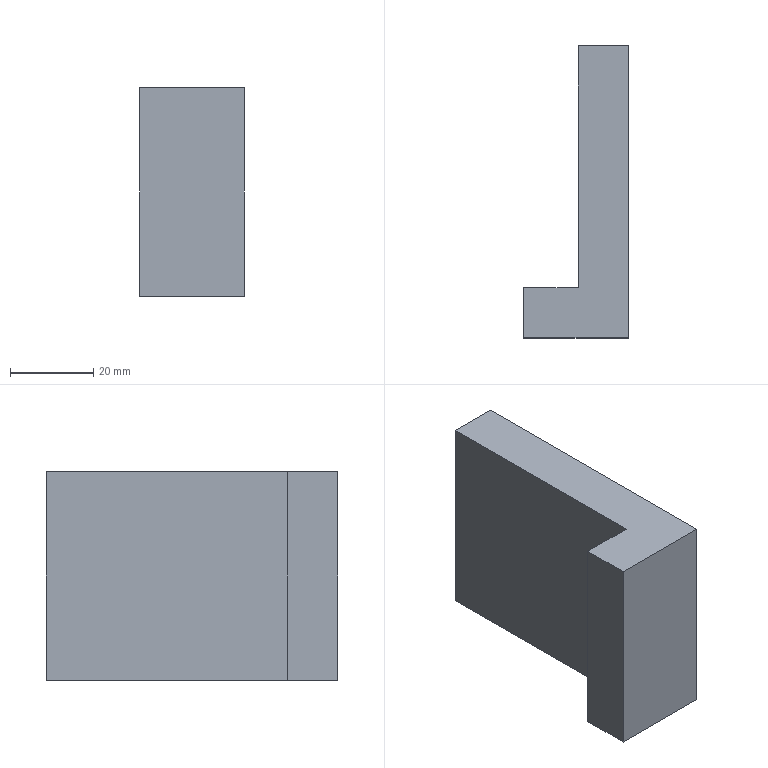Component | NX | CLAMP_PLATE_2 | 1 solid | 14 faces | box 25 x 70 x 50 mm | volume 49383 mm3 | plane 8 | cone 4 | cylinder 2 | commonest cylinder face diameters 5 x2
STEP:
#1=CARTESIAN_POINT('',(0.,0.,0.));
#2=DIRECTION('',(0.,0.,1.));
#3=DIRECTION('',(1.,0.,0.));
#4=AXIS2_PLACEMENT_3D('',#1,#2,#3);
#5=CARTESIAN_POINT('',(117.866,129.757,24.466));
#6=VERTEX_POINT('',#5);
#7=CARTESIAN_POINT('',(117.866,71.757,24.466));
#8=VERTEX_POINT('',#7);
#9=CARTESIAN_POINT('',(117.866,129.757,24.466));
#10=DIRECTION('',(-0.,-1.,0.));
#11=VECTOR('',#10,1.);
#12=LINE('',#9,#11);
#13=CARTESIAN_POINT('',(117.866,71.757,24.466));
#14=DIRECTION('',(-1.,0.,0.));
#15=DIRECTION('',(-0.,-1.,0.));
#16=AXIS2_PLACEMENT_3D('',#13,#14,#15);
#17=PLANE('',#16);
#18=CARTESIAN_POINT('',(-58.,0.));
#19=DIRECTION('',(1.,0.));
#20=VECTOR('',#19,1.);
#21=LINE('',#18,#20);
#22=(GEOMETRIC_REPRESENTATION_CONTEXT(2)PARAMETRIC_REPRESENTATION_CONTEXT()REPRESENTATION_CONTEXT('',''));
#23=DEFINITIONAL_REPRESENTATION('',(#21),#22);
#24=PCURVE('',#17,#23);
#25=CARTESIAN_POINT('',(129.866,59.757,24.466));
#26=DIRECTION('',(0.,0.,1.));
#27=DIRECTION('',(0.,1.,0.));
#28=AXIS2_PLACEMENT_3D('',#25,#26,#27);
#29=PLANE('',#28);
#30=CARTESIAN_POINT('',(70.,12.));
#31=DIRECTION('',(-1.,0.));
#32=VECTOR('',#31,1.);
#33=LINE('',#30,#32);
#34=(GEOMETRIC_REPRESENTATION_CONTEXT(2)PARAMETRIC_REPRESENTATION_CONTEXT()REPRESENTATION_CONTEXT('',''));
#35=DEFINITIONAL_REPRESENTATION('',(#33),#34);
#36=PCURVE('',#29,#35);
#37=SURFACE_CURVE('',#12,(#24,#36),.PCURVE_S1.);
#38=EDGE_CURVE('',#6,#8,#37,.T.);
#39=ORIENTED_EDGE('',*,*,#38,.T.);
#40=CARTESIAN_POINT('',(117.866,71.757,74.466));
#41=VERTEX_POINT('',#40);
#42=CARTESIAN_POINT('',(117.866,71.757,24.466));
#43=DIRECTION('',(0.,0.,1.));
#44=VECTOR('',#43,1.);
#45=LINE('',#42,#44);
#46=CARTESIAN_POINT('',(0.,0.));
#47=DIRECTION('',(0.,1.));
#48=VECTOR('',#47,1.);
#49=LINE('',#46,#48);
#50=(GEOMETRIC_REPRESENTATION_CONTEXT(2)PARAMETRIC_REPRESENTATION_CONTEXT()REPRESENTATION_CONTEXT('',''));
#51=DEFINITIONAL_REPRESENTATION('',(#49),#50);
#52=PCURVE('',#17,#51);
#53=CARTESIAN_POINT('',(117.866,71.757,24.466));
#54=DIRECTION('',(0.,1.,0.));
#55=DIRECTION('',(-1.,0.,0.));
#56=AXIS2_PLACEMENT_3D('',#53,#54,#55);
#57=PLANE('',#56);
#58=CARTESIAN_POINT('',(0.,0.));
#59=DIRECTION('',(0.,1.));
#60=VECTOR('',#59,1.);
#61=LINE('',#58,#60);
#62=(GEOMETRIC_REPRESENTATION_CONTEXT(2)PARAMETRIC_REPRESENTATION_CONTEXT()REPRESENTATION_CONTEXT('',''));
#63=DEFINITIONAL_REPRESENTATION('',(#61),#62);
#64=PCURVE('',#57,#63);
#65=SURFACE_CURVE('',#45,(#52,#64),.PCURVE_S1.);
#66=EDGE_CURVE('',#8,#41,#65,.T.);
#67=ORIENTED_EDGE('',*,*,#66,.T.);
#68=CARTESIAN_POINT('',(117.866,129.757,74.466));
#69=VERTEX_POINT('',#68);
#70=CARTESIAN_POINT('',(117.866,71.757,74.466));
#71=DIRECTION('',(-0.,-1.,0.));
#72=VECTOR('',#71,1.);
#73=LINE('',#70,#72);
#74=CARTESIAN_POINT('',(0.,50.));
#75=DIRECTION('',(1.,0.));
#76=VECTOR('',#75,1.);
#77=LINE('',#74,#76);
#78=(GEOMETRIC_REPRESENTATION_CONTEXT(2)PARAMETRIC_REPRESENTATION_CONTEXT()REPRESENTATION_CONTEXT('',''));
#79=DEFINITIONAL_REPRESENTATION('',(#77),#78);
#80=PCURVE('',#17,#79);
#81=CARTESIAN_POINT('',(129.866,59.757,74.466));
#82=DIRECTION('',(0.,0.,1.));
#83=DIRECTION('',(0.,1.,0.));
#84=AXIS2_PLACEMENT_3D('',#81,#82,#83);
#85=PLANE('',#84);
#86=CARTESIAN_POINT('',(12.,12.));
#87=DIRECTION('',(-1.,0.));
#88=VECTOR('',#87,1.);
#89=LINE('',#86,#88);
#90=(GEOMETRIC_REPRESENTATION_CONTEXT(2)PARAMETRIC_REPRESENTATION_CONTEXT()REPRESENTATION_CONTEXT('',''));
#91=DEFINITIONAL_REPRESENTATION('',(#89),#90);
#92=PCURVE('',#85,#91);
#93=SURFACE_CURVE('',#73,(#80,#92),.PCURVE_S1.);
#94=EDGE_CURVE('',#69,#41,#93,.T.);
#95=ORIENTED_EDGE('',*,*,#94,.F.);
#96=CARTESIAN_POINT('',(117.866,129.757,24.466));
#97=DIRECTION('',(0.,0.,1.));
#98=VECTOR('',#97,1.);
#99=LINE('',#96,#98);
#100=CARTESIAN_POINT('',(-58.,0.));
#101=DIRECTION('',(0.,1.));
#102=VECTOR('',#101,1.);
#103=LINE('',#100,#102);
#104=(GEOMETRIC_REPRESENTATION_CONTEXT(2)PARAMETRIC_REPRESENTATION_CONTEXT()REPRESENTATION_CONTEXT('',''));
#105=DEFINITIONAL_REPRESENTATION('',(#103),#104);
#106=PCURVE('',#17,#105);
#107=CARTESIAN_POINT('',(129.866,129.757,24.466));
#108=DIRECTION('',(0.,1.,0.));
#109=DIRECTION('',(-1.,0.,0.));
#110=AXIS2_PLACEMENT_3D('',#107,#108,#109);
#111=PLANE('',#110);
#112=CARTESIAN_POINT('',(12.,0.));
#113=DIRECTION('',(0.,1.));
#114=VECTOR('',#113,1.);
#115=LINE('',#112,#114);
#116=(GEOMETRIC_REPRESENTATION_CONTEXT(2)PARAMETRIC_REPRESENTATION_CONTEXT()REPRESENTATION_CONTEXT('',''));
#117=DEFINITIONAL_REPRESENTATION('',(#115),#116);
#118=PCURVE('',#111,#117);
#119=SURFACE_CURVE('',#99,(#106,#118),.PCURVE_S1.);
#120=EDGE_CURVE('',#6,#69,#119,.T.);
#121=ORIENTED_EDGE('',*,*,#120,.F.);
#122=EDGE_LOOP('',(#39,#67,#95,#121));
#123=FACE_BOUND('',#122,.T.);
#124=ADVANCED_FACE('',(#123),#17,.T.);
#125=CARTESIAN_POINT('',(104.866,59.757,74.466));
#126=VERTEX_POINT('',#125);
#127=CARTESIAN_POINT('',(129.866,59.757,74.466));
#128=VERTEX_POINT('',#127);
#129=CARTESIAN_POINT('',(117.866,59.757,74.466));
#130=DIRECTION('',(1.,-0.,0.));
#131=VECTOR('',#130,1.);
#132=LINE('',#129,#131);
#133=CARTESIAN_POINT('',(117.866,59.757,24.466));
#134=DIRECTION('',(-0.,-1.,0.));
#135=DIRECTION('',(1.,-0.,0.));
#136=AXIS2_PLACEMENT_3D('',#133,#134,#135);
#137=PLANE('',#136);
#138=CARTESIAN_POINT('',(0.,50.));
#139=DIRECTION('',(1.,0.));
#140=VECTOR('',#139,1.);
#141=LINE('',#138,#140);
#142=(GEOMETRIC_REPRESENTATION_CONTEXT(2)PARAMETRIC_REPRESENTATION_CONTEXT()REPRESENTATION_CONTEXT('',''));
#143=DEFINITIONAL_REPRESENTATION('',(#141),#142);
#144=PCURVE('',#137,#143);
#145=CARTESIAN_POINT('',(0.,12.));
#146=DIRECTION('',(-0.,-1.));
#147=VECTOR('',#146,1.);
#148=LINE('',#145,#147);
#149=(GEOMETRIC_REPRESENTATION_CONTEXT(2)PARAMETRIC_REPRESENTATION_CONTEXT()REPRESENTATION_CONTEXT('',''));
#150=DEFINITIONAL_REPRESENTATION('',(#148),#149);
#151=PCURVE('',#85,#150);
#152=SURFACE_CURVE('',#132,(#144,#151),.PCURVE_S1.);
#153=EDGE_CURVE('',#126,#128,#152,.T.);
#154=ORIENTED_EDGE('',*,*,#153,.F.);
#155=CARTESIAN_POINT('',(104.866,59.757,24.466));
#156=VERTEX_POINT('',#155);
#157=CARTESIAN_POINT('',(104.866,59.757,24.466));
#158=DIRECTION('',(0.,0.,1.));
#159=VECTOR('',#158,1.);
#160=LINE('',#157,#159);
#161=CARTESIAN_POINT('',(-13.,0.));
#162=DIRECTION('',(0.,1.));
#163=VECTOR('',#162,1.);
#164=LINE('',#161,#163);
#165=(GEOMETRIC_REPRESENTATION_CONTEXT(2)PARAMETRIC_REPRESENTATION_CONTEXT()REPRESENTATION_CONTEXT('',''));
#166=DEFINITIONAL_REPRESENTATION('',(#164),#165);
#167=PCURVE('',#137,#166);
#168=CARTESIAN_POINT('',(104.866,71.757,24.466));
#169=DIRECTION('',(-1.,0.,0.));
#170=DIRECTION('',(0.,0.,1.));
#171=AXIS2_PLACEMENT_3D('',#168,#169,#170);
#172=PLANE('',#171);
#173=CARTESIAN_POINT('',(0.,-12.));
#174=DIRECTION('',(1.,0.));
#175=VECTOR('',#174,1.);
#176=LINE('',#173,#175);
#177=(GEOMETRIC_REPRESENTATION_CONTEXT(2)PARAMETRIC_REPRESENTATION_CONTEXT()REPRESENTATION_CONTEXT('',''));
#178=DEFINITIONAL_REPRESENTATION('',(#176),#177);
#179=PCURVE('',#172,#178);
#180=SURFACE_CURVE('',#160,(#167,#179),.PCURVE_S1.);
#181=EDGE_CURVE('',#156,#126,#180,.T.);
#182=ORIENTED_EDGE('',*,*,#181,.F.);
#183=CARTESIAN_POINT('',(129.866,59.757,24.466));
#184=VERTEX_POINT('',#183);
#185=CARTESIAN_POINT('',(117.866,59.757,24.466));
#186=DIRECTION('',(1.,-0.,0.));
#187=VECTOR('',#186,1.);
#188=LINE('',#185,#187);
#189=CARTESIAN_POINT('',(0.,0.));
#190=DIRECTION('',(1.,0.));
#191=VECTOR('',#190,1.);
#192=LINE('',#189,#191);
#193=(GEOMETRIC_REPRESENTATION_CONTEXT(2)PARAMETRIC_REPRESENTATION_CONTEXT()REPRESENTATION_CONTEXT('',''));
#194=DEFINITIONAL_REPRESENTATION('',(#192),#193);
#195=PCURVE('',#137,#194);
#196=CARTESIAN_POINT('',(0.,12.));
#197=DIRECTION('',(-0.,-1.));
#198=VECTOR('',#197,1.);
#199=LINE('',#196,#198);
#200=(GEOMETRIC_REPRESENTATION_CONTEXT(2)PARAMETRIC_REPRESENTATION_CONTEXT()REPRESENTATION_CONTEXT('',''));
#201=DEFINITIONAL_REPRESENTATION('',(#199),#200);
#202=PCURVE('',#29,#201);
#203=SURFACE_CURVE('',#188,(#195,#202),.PCURVE_S1.);
#204=EDGE_CURVE('',#156,#184,#203,.T.);
#205=ORIENTED_EDGE('',*,*,#204,.T.);
#206=CARTESIAN_POINT('',(129.866,59.757,24.466));
#207=DIRECTION('',(0.,0.,1.));
#208=VECTOR('',#207,1.);
#209=LINE('',#206,#208);
#210=CARTESIAN_POINT('',(12.,0.));
#211=DIRECTION('',(0.,1.));
#212=VECTOR('',#211,1.);
#213=LINE('',#210,#212);
#214=(GEOMETRIC_REPRESENTATION_CONTEXT(2)PARAMETRIC_REPRESENTATION_CONTEXT()REPRESENTATION_CONTEXT('',''));
#215=DEFINITIONAL_REPRESENTATION('',(#213),#214);
#216=PCURVE('',#137,#215);
#217=CARTESIAN_POINT('',(129.866,59.757,24.466));
#218=DIRECTION('',(1.,0.,0.));
#219=DIRECTION('',(0.,0.,-1.));
#220=AXIS2_PLACEMENT_3D('',#217,#218,#219);
#221=PLANE('',#220);
#222=CARTESIAN_POINT('',(0.,-0.));
#223=DIRECTION('',(-1.,0.));
#224=VECTOR('',#223,1.);
#225=LINE('',#222,#224);
#226=(GEOMETRIC_REPRESENTATION_CONTEXT(2)PARAMETRIC_REPRESENTATION_CONTEXT()REPRESENTATION_CONTEXT('',''));
#227=DEFINITIONAL_REPRESENTATION('',(#225),#226);
#228=PCURVE('',#221,#227);
#229=SURFACE_CURVE('',#209,(#216,#228),.PCURVE_S1.);
#230=EDGE_CURVE('',#184,#128,#229,.T.);
#231=ORIENTED_EDGE('',*,*,#230,.T.);
#232=EDGE_LOOP('',(#154,#182,#205,#231));
#233=FACE_BOUND('',#232,.T.);
#234=ADVANCED_FACE('',(#233),#137,.T.);
#235=CARTESIAN_POINT('',(129.866,129.757,74.466));
#236=VERTEX_POINT('',#235);
#237=CARTESIAN_POINT('',(129.866,59.757,74.466));
#238=DIRECTION('',(0.,1.,0.));
#239=VECTOR('',#238,1.);
#240=LINE('',#237,#239);
#241=CARTESIAN_POINT('',(-50.,0.));
#242=DIRECTION('',(0.,1.));
#243=VECTOR('',#242,1.);
#244=LINE('',#241,#243);
#245=(GEOMETRIC_REPRESENTATION_CONTEXT(2)PARAMETRIC_REPRESENTATION_CONTEXT()REPRESENTATION_CONTEXT('',''));
#246=DEFINITIONAL_REPRESENTATION('',(#244),#245);
#247=PCURVE('',#221,#246);
#248=CARTESIAN_POINT('',(0.,0.));
#249=DIRECTION('',(1.,0.));
#250=VECTOR('',#249,1.);
#251=LINE('',#248,#250);
#252=(GEOMETRIC_REPRESENTATION_CONTEXT(2)PARAMETRIC_REPRESENTATION_CONTEXT()REPRESENTATION_CONTEXT('',''));
#253=DEFINITIONAL_REPRESENTATION('',(#251),#252);
#254=PCURVE('',#85,#253);
#255=SURFACE_CURVE('',#240,(#247,#254),.PCURVE_S1.);
#256=EDGE_CURVE('',#128,#236,#255,.T.);
#257=ORIENTED_EDGE('',*,*,#256,.F.);
#258=ORIENTED_EDGE('',*,*,#230,.F.);
#259=CARTESIAN_POINT('',(129.866,129.757,24.466));
#260=VERTEX_POINT('',#259);
#261=CARTESIAN_POINT('',(129.866,59.757,24.466));
#262=DIRECTION('',(0.,1.,0.));
#263=VECTOR('',#262,1.);
#264=LINE('',#261,#263);
#265=CARTESIAN_POINT('',(0.,0.));
#266=DIRECTION('',(0.,1.));
#267=VECTOR('',#266,1.);
#268=LINE('',#265,#267);
#269=(GEOMETRIC_REPRESENTATION_CONTEXT(2)PARAMETRIC_REPRESENTATION_CONTEXT()REPRESENTATION_CONTEXT('',''));
#270=DEFINITIONAL_REPRESENTATION('',(#268),#269);
#271=PCURVE('',#221,#270);
#272=CARTESIAN_POINT('',(0.,0.));
#273=DIRECTION('',(1.,0.));
#274=VECTOR('',#273,1.);
#275=LINE('',#272,#274);
#276=(GEOMETRIC_REPRESENTATION_CONTEXT(2)PARAMETRIC_REPRESENTATION_CONTEXT()REPRESENTATION_CONTEXT('',''));
#277=DEFINITIONAL_REPRESENTATION('',(#275),#276);
#278=PCURVE('',#29,#277);
#279=SURFACE_CURVE('',#264,(#271,#278),.PCURVE_S1.);
#280=EDGE_CURVE('',#184,#260,#279,.T.);
#281=ORIENTED_EDGE('',*,*,#280,.T.);
#282=CARTESIAN_POINT('',(129.866,129.757,24.466));
#283=DIRECTION('',(0.,0.,1.));
#284=VECTOR('',#283,1.);
#285=LINE('',#282,#284);
#286=CARTESIAN_POINT('',(0.,70.));
#287=DIRECTION('',(-1.,0.));
#288=VECTOR('',#287,1.);
#289=LINE('',#286,#288);
#290=(GEOMETRIC_REPRESENTATION_CONTEXT(2)PARAMETRIC_REPRESENTATION_CONTEXT()REPRESENTATION_CONTEXT('',''));
#291=DEFINITIONAL_REPRESENTATION('',(#289),#290);
#292=PCURVE('',#221,#291);
#293=CARTESIAN_POINT('',(0.,0.));
#294=DIRECTION('',(0.,1.));
#295=VECTOR('',#294,1.);
#296=LINE('',#293,#295);
#297=(GEOMETRIC_REPRESENTATION_CONTEXT(2)PARAMETRIC_REPRESENTATION_CONTEXT()REPRESENTATION_CONTEXT('',''));
#298=DEFINITIONAL_REPRESENTATION('',(#296),#297);
#299=PCURVE('',#111,#298);
#300=SURFACE_CURVE('',#285,(#292,#299),.PCURVE_S1.);
#301=EDGE_CURVE('',#260,#236,#300,.T.);
#302=ORIENTED_EDGE('',*,*,#301,.T.);
#303=EDGE_LOOP('',(#257,#258,#281,#302));
#304=FACE_BOUND('',#303,.T.);
#305=ADVANCED_FACE('',(#304),#221,.T.);
#306=CARTESIAN_POINT('',(120.866,129.757,34.466));
#307=VERTEX_POINT('',#306);
#308=CARTESIAN_POINT('',(123.866,129.757,34.466));
#309=DIRECTION('',(-0.,-1.,0.));
#310=DIRECTION('',(-1.,0.,0.));
#311=AXIS2_PLACEMENT_3D('',#308,#309,#310);
#312=CIRCLE('',#311,3.);
#313=CARTESIAN_POINT('',(9.,10.));
#314=CARTESIAN_POINT('',(9.,4.804));
#315=CARTESIAN_POINT('',(4.5,7.402));
#316=CARTESIAN_POINT('',(0.,10.));
#317=CARTESIAN_POINT('',(4.5,12.598));
#318=CARTESIAN_POINT('',(9.,15.196));
#319=CARTESIAN_POINT('',(9.,10.));
#320=(BOUNDED_CURVE()B_SPLINE_CURVE(2,(#313,#314,#315,#316,#317,#318,#319),.UNSPECIFIED.,.T.,.F.)B_SPLINE_CURVE_WITH_KNOTS((1,2,2,2,2,1),(-2.094,0.,2.094,4.189,6.283,8.378),.UNSPECIFIED.)CURVE()GEOMETRIC_REPRESENTATION_ITEM()RATIONAL_B_SPLINE_CURVE((1.,0.5,1.,0.5,1.,0.5,1.))REPRESENTATION_ITEM(''));
#321=(GEOMETRIC_REPRESENTATION_CONTEXT(2)PARAMETRIC_REPRESENTATION_CONTEXT()REPRESENTATION_CONTEXT('',''));
#322=DEFINITIONAL_REPRESENTATION('',(#320),#321);
#323=PCURVE('',#111,#322);
#324=CARTESIAN_POINT('',(123.866,129.757,34.466));
#325=DIRECTION('',(0.,1.,0.));
#326=DIRECTION('',(-1.,0.,0.));
#327=AXIS2_PLACEMENT_3D('',#324,#325,#326);
#328=CONICAL_SURFACE('',#327,3.,0.7854);
#329=CARTESIAN_POINT('',(6.283,-0.));
#330=DIRECTION('',(-1.,0.));
#331=VECTOR('',#330,1.);
#332=LINE('',#329,#331);
#333=(GEOMETRIC_REPRESENTATION_CONTEXT(2)PARAMETRIC_REPRESENTATION_CONTEXT()REPRESENTATION_CONTEXT('',''));
#334=DEFINITIONAL_REPRESENTATION('',(#332),#333);
#335=PCURVE('',#328,#334);
#336=SURFACE_CURVE('',#312,(#323,#335),.PCURVE_S1.);
#337=EDGE_CURVE('',#307,#307,#336,.T.);
#338=ORIENTED_EDGE('',*,*,#337,.T.);
#339=EDGE_LOOP('',(#338));
#340=FACE_BOUND('',#339,.T.);
#341=CARTESIAN_POINT('',(120.866,129.757,64.466));
#342=VERTEX_POINT('',#341);
#343=CARTESIAN_POINT('',(123.866,129.757,64.466));
#344=DIRECTION('',(-0.,-1.,0.));
#345=DIRECTION('',(-1.,0.,0.));
#346=AXIS2_PLACEMENT_3D('',#343,#344,#345);
#347=CIRCLE('',#346,3.);
#348=CARTESIAN_POINT('',(9.,40.));
#349=CARTESIAN_POINT('',(9.,34.804));
#350=CARTESIAN_POINT('',(4.5,37.402));
#351=CARTESIAN_POINT('',(0.,40.));
#352=CARTESIAN_POINT('',(4.5,42.598));
#353=CARTESIAN_POINT('',(9.,45.196));
#354=CARTESIAN_POINT('',(9.,40.));
#355=(BOUNDED_CURVE()B_SPLINE_CURVE(2,(#348,#349,#350,#351,#352,#353,#354),.UNSPECIFIED.,.T.,.F.)B_SPLINE_CURVE_WITH_KNOTS((1,2,2,2,2,1),(-2.094,0.,2.094,4.189,6.283,8.378),.UNSPECIFIED.)CURVE()GEOMETRIC_REPRESENTATION_ITEM()RATIONAL_B_SPLINE_CURVE((1.,0.5,1.,0.5,1.,0.5,1.))REPRESENTATION_ITEM(''));
#356=(GEOMETRIC_REPRESENTATION_CONTEXT(2)PARAMETRIC_REPRESENTATION_CONTEXT()REPRESENTATION_CONTEXT('',''));
#357=DEFINITIONAL_REPRESENTATION('',(#355),#356);
#358=PCURVE('',#111,#357);
#359=CARTESIAN_POINT('',(123.866,129.757,64.466));
#360=DIRECTION('',(0.,1.,0.));
#361=DIRECTION('',(-1.,0.,0.));
#362=AXIS2_PLACEMENT_3D('',#359,#360,#361);
#363=CONICAL_SURFACE('',#362,3.,0.7854);
#364=CARTESIAN_POINT('',(6.283,-0.));
#365=DIRECTION('',(-1.,0.));
#366=VECTOR('',#365,1.);
#367=LINE('',#364,#366);
#368=(GEOMETRIC_REPRESENTATION_CONTEXT(2)PARAMETRIC_REPRESENTATION_CONTEXT()REPRESENTATION_CONTEXT('',''));
#369=DEFINITIONAL_REPRESENTATION('',(#367),#368);
#370=PCURVE('',#363,#369);
#371=SURFACE_CURVE('',#347,(#358,#370),.PCURVE_S1.);
#372=EDGE_CURVE('',#342,#342,#371,.T.);
#373=ORIENTED_EDGE('',*,*,#372,.T.);
#374=EDGE_LOOP('',(#373));
#375=FACE_BOUND('',#374,.T.);
#376=CARTESIAN_POINT('',(129.866,129.757,74.466));
#377=DIRECTION('',(-1.,0.,0.));
#378=VECTOR('',#377,1.);
#379=LINE('',#376,#378);
#380=CARTESIAN_POINT('',(0.,50.));
#381=DIRECTION('',(1.,0.));
#382=VECTOR('',#381,1.);
#383=LINE('',#380,#382);
#384=(GEOMETRIC_REPRESENTATION_CONTEXT(2)PARAMETRIC_REPRESENTATION_CONTEXT()REPRESENTATION_CONTEXT('',''));
#385=DEFINITIONAL_REPRESENTATION('',(#383),#384);
#386=PCURVE('',#111,#385);
#387=CARTESIAN_POINT('',(70.,0.));
#388=DIRECTION('',(0.,1.));
#389=VECTOR('',#388,1.);
#390=LINE('',#387,#389);
#391=(GEOMETRIC_REPRESENTATION_CONTEXT(2)PARAMETRIC_REPRESENTATION_CONTEXT()REPRESENTATION_CONTEXT('',''));
#392=DEFINITIONAL_REPRESENTATION('',(#390),#391);
#393=PCURVE('',#85,#392);
#394=SURFACE_CURVE('',#379,(#386,#393),.PCURVE_S1.);
#395=EDGE_CURVE('',#236,#69,#394,.T.);
#396=ORIENTED_EDGE('',*,*,#395,.F.);
#397=ORIENTED_EDGE('',*,*,#301,.F.);
#398=CARTESIAN_POINT('',(129.866,129.757,24.466));
#399=DIRECTION('',(-1.,0.,0.));
#400=VECTOR('',#399,1.);
#401=LINE('',#398,#400);
#402=CARTESIAN_POINT('',(0.,0.));
#403=DIRECTION('',(1.,0.));
#404=VECTOR('',#403,1.);
#405=LINE('',#402,#404);
#406=(GEOMETRIC_REPRESENTATION_CONTEXT(2)PARAMETRIC_REPRESENTATION_CONTEXT()REPRESENTATION_CONTEXT('',''));
#407=DEFINITIONAL_REPRESENTATION('',(#405),#406);
#408=PCURVE('',#111,#407);
#409=CARTESIAN_POINT('',(70.,0.));
#410=DIRECTION('',(0.,1.));
#411=VECTOR('',#410,1.);
#412=LINE('',#409,#411);
#413=(GEOMETRIC_REPRESENTATION_CONTEXT(2)PARAMETRIC_REPRESENTATION_CONTEXT()REPRESENTATION_CONTEXT('',''));
#414=DEFINITIONAL_REPRESENTATION('',(#412),#413);
#415=PCURVE('',#29,#414);
#416=SURFACE_CURVE('',#401,(#408,#415),.PCURVE_S1.);
#417=EDGE_CURVE('',#260,#6,#416,.T.);
#418=ORIENTED_EDGE('',*,*,#417,.T.);
#419=ORIENTED_EDGE('',*,*,#120,.T.);
#420=EDGE_LOOP('',(#396,#397,#418,#419));
#421=FACE_BOUND('',#420,.T.);
#422=ADVANCED_FACE('',(#340,#375,#421),#111,.T.);
#423=ORIENTED_EDGE('',*,*,#204,.F.);
#424=CARTESIAN_POINT('',(104.866,71.757,24.466));
#425=VERTEX_POINT('',#424);
#426=CARTESIAN_POINT('',(104.866,71.757,24.466));
#427=DIRECTION('',(0.,-1.,0.));
#428=VECTOR('',#427,1.);
#429=LINE('',#426,#428);
#430=CARTESIAN_POINT('',(12.,25.));
#431=DIRECTION('',(-1.,0.));
#432=VECTOR('',#431,1.);
#433=LINE('',#430,#432);
#434=(GEOMETRIC_REPRESENTATION_CONTEXT(2)PARAMETRIC_REPRESENTATION_CONTEXT()REPRESENTATION_CONTEXT('',''));
#435=DEFINITIONAL_REPRESENTATION('',(#433),#434);
#436=PCURVE('',#29,#435);
#437=CARTESIAN_POINT('',(0.,0.));
#438=DIRECTION('',(0.,-1.));
#439=VECTOR('',#438,1.);
#440=LINE('',#437,#439);
#441=(GEOMETRIC_REPRESENTATION_CONTEXT(2)PARAMETRIC_REPRESENTATION_CONTEXT()REPRESENTATION_CONTEXT('',''));
#442=DEFINITIONAL_REPRESENTATION('',(#440),#441);
#443=PCURVE('',#172,#442);
#444=SURFACE_CURVE('',#429,(#436,#443),.PCURVE_S1.);
#445=EDGE_CURVE('',#425,#156,#444,.T.);
#446=ORIENTED_EDGE('',*,*,#445,.F.);
#447=CARTESIAN_POINT('',(117.866,71.757,24.466));
#448=DIRECTION('',(-1.,0.,0.));
#449=VECTOR('',#448,1.);
#450=LINE('',#447,#449);
#451=CARTESIAN_POINT('',(12.,12.));
#452=DIRECTION('',(0.,1.));
#453=VECTOR('',#452,1.);
#454=LINE('',#451,#453);
#455=(GEOMETRIC_REPRESENTATION_CONTEXT(2)PARAMETRIC_REPRESENTATION_CONTEXT()REPRESENTATION_CONTEXT('',''));
#456=DEFINITIONAL_REPRESENTATION('',(#454),#455);
#457=PCURVE('',#29,#456);
#458=CARTESIAN_POINT('',(0.,0.));
#459=DIRECTION('',(1.,0.));
#460=VECTOR('',#459,1.);
#461=LINE('',#458,#460);
#462=(GEOMETRIC_REPRESENTATION_CONTEXT(2)PARAMETRIC_REPRESENTATION_CONTEXT()REPRESENTATION_CONTEXT('',''));
#463=DEFINITIONAL_REPRESENTATION('',(#461),#462);
#464=PCURVE('',#57,#463);
#465=SURFACE_CURVE('',#450,(#457,#464),.PCURVE_S1.);
#466=EDGE_CURVE('',#8,#425,#465,.T.);
#467=ORIENTED_EDGE('',*,*,#466,.F.);
#468=ORIENTED_EDGE('',*,*,#38,.F.);
#469=ORIENTED_EDGE('',*,*,#417,.F.);
#470=ORIENTED_EDGE('',*,*,#280,.F.);
#471=EDGE_LOOP('',(#423,#446,#467,#468,#469,#470));
#472=FACE_BOUND('',#471,.T.);
#473=ADVANCED_FACE('',(#472),#29,.F.);
#474=ORIENTED_EDGE('',*,*,#153,.T.);
#475=ORIENTED_EDGE('',*,*,#256,.T.);
#476=ORIENTED_EDGE('',*,*,#395,.T.);
#477=ORIENTED_EDGE('',*,*,#94,.T.);
#478=CARTESIAN_POINT('',(104.866,71.757,74.466));
#479=VERTEX_POINT('',#478);
#480=CARTESIAN_POINT('',(117.866,71.757,74.466));
#481=DIRECTION('',(-1.,0.,0.));
#482=VECTOR('',#481,1.);
#483=LINE('',#480,#482);
#484=CARTESIAN_POINT('',(12.,12.));
#485=DIRECTION('',(0.,1.));
#486=VECTOR('',#485,1.);
#487=LINE('',#484,#486);
#488=(GEOMETRIC_REPRESENTATION_CONTEXT(2)PARAMETRIC_REPRESENTATION_CONTEXT()REPRESENTATION_CONTEXT('',''));
#489=DEFINITIONAL_REPRESENTATION('',(#487),#488);
#490=PCURVE('',#85,#489);
#491=CARTESIAN_POINT('',(0.,50.));
#492=DIRECTION('',(1.,0.));
#493=VECTOR('',#492,1.);
#494=LINE('',#491,#493);
#495=(GEOMETRIC_REPRESENTATION_CONTEXT(2)PARAMETRIC_REPRESENTATION_CONTEXT()REPRESENTATION_CONTEXT('',''));
#496=DEFINITIONAL_REPRESENTATION('',(#494),#495);
#497=PCURVE('',#57,#496);
#498=SURFACE_CURVE('',#483,(#490,#497),.PCURVE_S1.);
#499=EDGE_CURVE('',#41,#479,#498,.T.);
#500=ORIENTED_EDGE('',*,*,#499,.T.);
#501=CARTESIAN_POINT('',(104.866,71.757,74.466));
#502=DIRECTION('',(0.,-1.,0.));
#503=VECTOR('',#502,1.);
#504=LINE('',#501,#503);
#505=CARTESIAN_POINT('',(12.,25.));
#506=DIRECTION('',(-1.,0.));
#507=VECTOR('',#506,1.);
#508=LINE('',#505,#507);
#509=(GEOMETRIC_REPRESENTATION_CONTEXT(2)PARAMETRIC_REPRESENTATION_CONTEXT()REPRESENTATION_CONTEXT('',''));
#510=DEFINITIONAL_REPRESENTATION('',(#508),#509);
#511=PCURVE('',#85,#510);
#512=CARTESIAN_POINT('',(50.,0.));
#513=DIRECTION('',(0.,-1.));
#514=VECTOR('',#513,1.);
#515=LINE('',#512,#514);
#516=(GEOMETRIC_REPRESENTATION_CONTEXT(2)PARAMETRIC_REPRESENTATION_CONTEXT()REPRESENTATION_CONTEXT('',''));
#517=DEFINITIONAL_REPRESENTATION('',(#515),#516);
#518=PCURVE('',#172,#517);
#519=SURFACE_CURVE('',#504,(#511,#518),.PCURVE_S1.);
#520=EDGE_CURVE('',#479,#126,#519,.T.);
#521=ORIENTED_EDGE('',*,*,#520,.T.);
#522=EDGE_LOOP('',(#474,#475,#476,#477,#500,#521));
#523=FACE_BOUND('',#522,.T.);
#524=ADVANCED_FACE('',(#523),#85,.T.);
#525=ORIENTED_EDGE('',*,*,#499,.F.);
#526=ORIENTED_EDGE('',*,*,#66,.F.);
#527=ORIENTED_EDGE('',*,*,#466,.T.);
#528=CARTESIAN_POINT('',(104.866,71.757,24.466));
#529=DIRECTION('',(0.,0.,1.));
#530=VECTOR('',#529,1.);
#531=LINE('',#528,#530);
#532=CARTESIAN_POINT('',(13.,0.));
#533=DIRECTION('',(0.,1.));
#534=VECTOR('',#533,1.);
#535=LINE('',#532,#534);
#536=(GEOMETRIC_REPRESENTATION_CONTEXT(2)PARAMETRIC_REPRESENTATION_CONTEXT()REPRESENTATION_CONTEXT('',''));
#537=DEFINITIONAL_REPRESENTATION('',(#535),#536);
#538=PCURVE('',#57,#537);
#539=CARTESIAN_POINT('',(0.,0.));
#540=DIRECTION('',(1.,0.));
#541=VECTOR('',#540,1.);
#542=LINE('',#539,#541);
#543=(GEOMETRIC_REPRESENTATION_CONTEXT(2)PARAMETRIC_REPRESENTATION_CONTEXT()REPRESENTATION_CONTEXT('',''));
#544=DEFINITIONAL_REPRESENTATION('',(#542),#543);
#545=PCURVE('',#172,#544);
#546=SURFACE_CURVE('',#531,(#538,#545),.PCURVE_S1.);
#547=EDGE_CURVE('',#425,#479,#546,.T.);
#548=ORIENTED_EDGE('',*,*,#547,.T.);
#549=EDGE_LOOP('',(#525,#526,#527,#548));
#550=FACE_BOUND('',#549,.T.);
#551=ADVANCED_FACE('',(#550),#57,.T.);
#552=ORIENTED_EDGE('',*,*,#520,.F.);
#553=ORIENTED_EDGE('',*,*,#547,.F.);
#554=ORIENTED_EDGE('',*,*,#445,.T.);
#555=ORIENTED_EDGE('',*,*,#181,.T.);
#556=EDGE_LOOP('',(#552,#553,#554,#555));
#557=FACE_BOUND('',#556,.T.);
#558=ADVANCED_FACE('',(#557),#172,.T.);
#559=CARTESIAN_POINT('',(121.366,119.757,64.466));
#560=VERTEX_POINT('',#559);
#561=CARTESIAN_POINT('',(126.366,119.757,64.466));
#562=VERTEX_POINT('',#561);
#563=CARTESIAN_POINT('',(123.866,119.757,64.466));
#564=DIRECTION('',(0.,1.,0.));
#565=DIRECTION('',(1.,-0.,0.));
#566=AXIS2_PLACEMENT_3D('',#563,#564,#565);
#567=CIRCLE('',#566,2.5);
#568=CARTESIAN_POINT('',(123.866,119.757,64.466));
#569=DIRECTION('',(0.,1.,0.));
#570=DIRECTION('',(-1.,0.,0.));
#571=AXIS2_PLACEMENT_3D('',#568,#569,#570);
#572=CONICAL_SURFACE('',#571,2.5,1.03);
#573=CARTESIAN_POINT('',(-3.142,0.));
#574=DIRECTION('',(1.,0.));
#575=VECTOR('',#574,1.);
#576=LINE('',#573,#575);
#577=(GEOMETRIC_REPRESENTATION_CONTEXT(2)PARAMETRIC_REPRESENTATION_CONTEXT()REPRESENTATION_CONTEXT('',''));
#578=DEFINITIONAL_REPRESENTATION('',(#576),#577);
#579=PCURVE('',#572,#578);
#580=CARTESIAN_POINT('',(123.866,129.757,64.466));
#581=DIRECTION('',(-0.,-1.,0.));
#582=DIRECTION('',(1.,-0.,0.));
#583=AXIS2_PLACEMENT_3D('',#580,#581,#582);
#584=CYLINDRICAL_SURFACE('',#583,2.5);
#585=CARTESIAN_POINT('',(12.566,10.));
#586=DIRECTION('',(-1.,0.));
#587=VECTOR('',#586,1.);
#588=LINE('',#585,#587);
#589=(GEOMETRIC_REPRESENTATION_CONTEXT(2)PARAMETRIC_REPRESENTATION_CONTEXT()REPRESENTATION_CONTEXT('',''));
#590=DEFINITIONAL_REPRESENTATION('',(#588),#589);
#591=PCURVE('',#584,#590);
#592=SURFACE_CURVE('',#567,(#579,#591),.PCURVE_S1.);
#593=EDGE_CURVE('',#560,#562,#592,.T.);
#594=ORIENTED_EDGE('',*,*,#593,.F.);
#595=CARTESIAN_POINT('',(123.866,118.255,64.466));
#596=VERTEX_POINT('',#595);
#597=CARTESIAN_POINT('',(123.866,118.255,64.466));
#598=CARTESIAN_POINT('',(121.366,119.757,64.466));
#599=B_SPLINE_CURVE_WITH_KNOTS('',1,(#597,#598),.UNSPECIFIED.,.F.,.F.,(2,2),(-2.917,0.),.PIECEWISE_BEZIER_KNOTS.);
#600=CARTESIAN_POINT('',(0.,0.));
#601=DIRECTION('',(0.,1.));
#602=VECTOR('',#601,1.);
#603=LINE('',#600,#602);
#604=(GEOMETRIC_REPRESENTATION_CONTEXT(2)PARAMETRIC_REPRESENTATION_CONTEXT()REPRESENTATION_CONTEXT('',''));
#605=DEFINITIONAL_REPRESENTATION('',(#603),#604);
#606=PCURVE('',#572,#605);
#607=CARTESIAN_POINT('',(6.283,0.));
#608=DIRECTION('',(0.,1.));
#609=VECTOR('',#608,1.);
#610=LINE('',#607,#609);
#611=(GEOMETRIC_REPRESENTATION_CONTEXT(2)PARAMETRIC_REPRESENTATION_CONTEXT()REPRESENTATION_CONTEXT('',''));
#612=DEFINITIONAL_REPRESENTATION('',(#610),#611);
#613=PCURVE('',#572,#612);
#614=SEAM_CURVE('',#599,(#606,#613),.PCURVE_S1.);
#615=EDGE_CURVE('',#596,#560,#614,.T.);
#616=ORIENTED_EDGE('',*,*,#615,.F.);
#617=ORIENTED_EDGE('',*,*,#615,.T.);
#618=CARTESIAN_POINT('',(123.866,119.757,64.466));
#619=DIRECTION('',(0.,1.,0.));
#620=DIRECTION('',(1.,-0.,0.));
#621=AXIS2_PLACEMENT_3D('',#618,#619,#620);
#622=CIRCLE('',#621,2.5);
#623=CARTESIAN_POINT('',(3.142,0.));
#624=DIRECTION('',(1.,0.));
#625=VECTOR('',#624,1.);
#626=LINE('',#623,#625);
#627=(GEOMETRIC_REPRESENTATION_CONTEXT(2)PARAMETRIC_REPRESENTATION_CONTEXT()REPRESENTATION_CONTEXT('',''));
#628=DEFINITIONAL_REPRESENTATION('',(#626),#627);
#629=PCURVE('',#572,#628);
#630=CARTESIAN_POINT('',(6.283,10.));
#631=DIRECTION('',(-1.,0.));
#632=VECTOR('',#631,1.);
#633=LINE('',#630,#632);
#634=(GEOMETRIC_REPRESENTATION_CONTEXT(2)PARAMETRIC_REPRESENTATION_CONTEXT()REPRESENTATION_CONTEXT('',''));
#635=DEFINITIONAL_REPRESENTATION('',(#633),#634);
#636=PCURVE('',#584,#635);
#637=SURFACE_CURVE('',#622,(#629,#636),.PCURVE_S1.);
#638=EDGE_CURVE('',#562,#560,#637,.T.);
#639=ORIENTED_EDGE('',*,*,#638,.F.);
#640=EDGE_LOOP('',(#594,#616,#617,#639));
#641=FACE_BOUND('',#640,.F.);
#642=ADVANCED_FACE('',(#641),#572,.F.);
#643=CARTESIAN_POINT('',(121.366,129.257,64.466));
#644=VERTEX_POINT('',#643);
#645=CARTESIAN_POINT('',(123.866,129.257,64.466));
#646=DIRECTION('',(0.,1.,0.));
#647=DIRECTION('',(-1.,0.,0.));
#648=AXIS2_PLACEMENT_3D('',#645,#646,#647);
#649=CIRCLE('',#648,2.5);
#650=CARTESIAN_POINT('',(9.425,0.5));
#651=DIRECTION('',(-1.,0.));
#652=VECTOR('',#651,1.);
#653=LINE('',#650,#652);
#654=(GEOMETRIC_REPRESENTATION_CONTEXT(2)PARAMETRIC_REPRESENTATION_CONTEXT()REPRESENTATION_CONTEXT('',''));
#655=DEFINITIONAL_REPRESENTATION('',(#653),#654);
#656=PCURVE('',#584,#655);
#657=CARTESIAN_POINT('',(0.,-0.5));
#658=DIRECTION('',(1.,0.));
#659=VECTOR('',#658,1.);
#660=LINE('',#657,#659);
#661=(GEOMETRIC_REPRESENTATION_CONTEXT(2)PARAMETRIC_REPRESENTATION_CONTEXT()REPRESENTATION_CONTEXT('',''));
#662=DEFINITIONAL_REPRESENTATION('',(#660),#661);
#663=PCURVE('',#363,#662);
#664=SURFACE_CURVE('',#649,(#656,#663),.PCURVE_S1.);
#665=EDGE_CURVE('',#644,#644,#664,.T.);
#666=ORIENTED_EDGE('',*,*,#665,.F.);
#667=CARTESIAN_POINT('',(121.366,129.257,64.466));
#668=CARTESIAN_POINT('',(121.366,119.757,64.466));
#669=B_SPLINE_CURVE_WITH_KNOTS('',1,(#667,#668),.UNSPECIFIED.,.F.,.F.,(2,2),(0.5,10.),.PIECEWISE_BEZIER_KNOTS.);
#670=CARTESIAN_POINT('',(9.425,0.));
#671=DIRECTION('',(0.,1.));
#672=VECTOR('',#671,1.);
#673=LINE('',#670,#672);
#674=(GEOMETRIC_REPRESENTATION_CONTEXT(2)PARAMETRIC_REPRESENTATION_CONTEXT()REPRESENTATION_CONTEXT('',''));
#675=DEFINITIONAL_REPRESENTATION('',(#673),#674);
#676=PCURVE('',#584,#675);
#677=CARTESIAN_POINT('',(3.142,0.));
#678=DIRECTION('',(0.,1.));
#679=VECTOR('',#678,1.);
#680=LINE('',#677,#679);
#681=(GEOMETRIC_REPRESENTATION_CONTEXT(2)PARAMETRIC_REPRESENTATION_CONTEXT()REPRESENTATION_CONTEXT('',''));
#682=DEFINITIONAL_REPRESENTATION('',(#680),#681);
#683=PCURVE('',#584,#682);
#684=SEAM_CURVE('',#669,(#676,#683),.PCURVE_S1.);
#685=EDGE_CURVE('',#644,#560,#684,.T.);
#686=ORIENTED_EDGE('',*,*,#685,.T.);
#687=ORIENTED_EDGE('',*,*,#593,.T.);
#688=ORIENTED_EDGE('',*,*,#638,.T.);
#689=ORIENTED_EDGE('',*,*,#685,.F.);
#690=EDGE_LOOP('',(#666,#686,#687,#688,#689));
#691=FACE_BOUND('',#690,.F.);
#692=ADVANCED_FACE('',(#691),#584,.F.);
#693=ORIENTED_EDGE('',*,*,#665,.T.);
#694=CARTESIAN_POINT('',(121.366,129.257,64.466));
#695=CARTESIAN_POINT('',(120.866,129.757,64.466));
#696=B_SPLINE_CURVE_WITH_KNOTS('',1,(#694,#695),.UNSPECIFIED.,.F.,.F.,(2,2),(-0.7071,-0.),.PIECEWISE_BEZIER_KNOTS.);
#697=CARTESIAN_POINT('',(6.283,0.));
#698=DIRECTION('',(0.,1.));
#699=VECTOR('',#698,1.);
#700=LINE('',#697,#699);
#701=(GEOMETRIC_REPRESENTATION_CONTEXT(2)PARAMETRIC_REPRESENTATION_CONTEXT()REPRESENTATION_CONTEXT('',''));
#702=DEFINITIONAL_REPRESENTATION('',(#700),#701);
#703=PCURVE('',#363,#702);
#704=CARTESIAN_POINT('',(0.,0.));
#705=DIRECTION('',(0.,1.));
#706=VECTOR('',#705,1.);
#707=LINE('',#704,#706);
#708=(GEOMETRIC_REPRESENTATION_CONTEXT(2)PARAMETRIC_REPRESENTATION_CONTEXT()REPRESENTATION_CONTEXT('',''));
#709=DEFINITIONAL_REPRESENTATION('',(#707),#708);
#710=PCURVE('',#363,#709);
#711=SEAM_CURVE('',#696,(#703,#710),.PCURVE_S1.);
#712=EDGE_CURVE('',#644,#342,#711,.T.);
#713=ORIENTED_EDGE('',*,*,#712,.T.);
#714=ORIENTED_EDGE('',*,*,#372,.T.);
#715=ORIENTED_EDGE('',*,*,#712,.F.);
#716=EDGE_LOOP('',(#693,#713,#714,#715));
#717=FACE_BOUND('',#716,.F.);
#718=ADVANCED_FACE('',(#717),#363,.F.);
#719=CARTESIAN_POINT('',(121.366,119.757,34.466));
#720=VERTEX_POINT('',#719);
#721=CARTESIAN_POINT('',(126.366,119.757,34.466));
#722=VERTEX_POINT('',#721);
#723=CARTESIAN_POINT('',(123.866,119.757,34.466));
#724=DIRECTION('',(0.,1.,0.));
#725=DIRECTION('',(1.,-0.,0.));
#726=AXIS2_PLACEMENT_3D('',#723,#724,#725);
#727=CIRCLE('',#726,2.5);
#728=CARTESIAN_POINT('',(123.866,119.757,34.466));
#729=DIRECTION('',(0.,1.,0.));
#730=DIRECTION('',(-1.,0.,0.));
#731=AXIS2_PLACEMENT_3D('',#728,#729,#730);
#732=CONICAL_SURFACE('',#731,2.5,1.03);
#733=CARTESIAN_POINT('',(-3.142,0.));
#734=DIRECTION('',(1.,0.));
#735=VECTOR('',#734,1.);
#736=LINE('',#733,#735);
#737=(GEOMETRIC_REPRESENTATION_CONTEXT(2)PARAMETRIC_REPRESENTATION_CONTEXT()REPRESENTATION_CONTEXT('',''));
#738=DEFINITIONAL_REPRESENTATION('',(#736),#737);
#739=PCURVE('',#732,#738);
#740=CARTESIAN_POINT('',(123.866,129.757,34.466));
#741=DIRECTION('',(-0.,-1.,0.));
#742=DIRECTION('',(1.,-0.,0.));
#743=AXIS2_PLACEMENT_3D('',#740,#741,#742);
#744=CYLINDRICAL_SURFACE('',#743,2.5);
#745=CARTESIAN_POINT('',(12.566,10.));
#746=DIRECTION('',(-1.,0.));
#747=VECTOR('',#746,1.);
#748=LINE('',#745,#747);
#749=(GEOMETRIC_REPRESENTATION_CONTEXT(2)PARAMETRIC_REPRESENTATION_CONTEXT()REPRESENTATION_CONTEXT('',''));
#750=DEFINITIONAL_REPRESENTATION('',(#748),#749);
#751=PCURVE('',#744,#750);
#752=SURFACE_CURVE('',#727,(#739,#751),.PCURVE_S1.);
#753=EDGE_CURVE('',#720,#722,#752,.T.);
#754=ORIENTED_EDGE('',*,*,#753,.F.);
#755=CARTESIAN_POINT('',(123.866,118.255,34.466));
#756=VERTEX_POINT('',#755);
#757=CARTESIAN_POINT('',(123.866,118.255,34.466));
#758=CARTESIAN_POINT('',(121.366,119.757,34.466));
#759=B_SPLINE_CURVE_WITH_KNOTS('',1,(#757,#758),.UNSPECIFIED.,.F.,.F.,(2,2),(-2.917,0.),.PIECEWISE_BEZIER_KNOTS.);
#760=CARTESIAN_POINT('',(0.,0.));
#761=DIRECTION('',(0.,1.));
#762=VECTOR('',#761,1.);
#763=LINE('',#760,#762);
#764=(GEOMETRIC_REPRESENTATION_CONTEXT(2)PARAMETRIC_REPRESENTATION_CONTEXT()REPRESENTATION_CONTEXT('',''));
#765=DEFINITIONAL_REPRESENTATION('',(#763),#764);
#766=PCURVE('',#732,#765);
#767=CARTESIAN_POINT('',(6.283,0.));
#768=DIRECTION('',(0.,1.));
#769=VECTOR('',#768,1.);
#770=LINE('',#767,#769);
#771=(GEOMETRIC_REPRESENTATION_CONTEXT(2)PARAMETRIC_REPRESENTATION_CONTEXT()REPRESENTATION_CONTEXT('',''));
#772=DEFINITIONAL_REPRESENTATION('',(#770),#771);
#773=PCURVE('',#732,#772);
#774=SEAM_CURVE('',#759,(#766,#773),.PCURVE_S1.);
#775=EDGE_CURVE('',#756,#720,#774,.T.);
#776=ORIENTED_EDGE('',*,*,#775,.F.);
#777=ORIENTED_EDGE('',*,*,#775,.T.);
#778=CARTESIAN_POINT('',(123.866,119.757,34.466));
#779=DIRECTION('',(0.,1.,0.));
#780=DIRECTION('',(1.,-0.,0.));
#781=AXIS2_PLACEMENT_3D('',#778,#779,#780);
#782=CIRCLE('',#781,2.5);
#783=CARTESIAN_POINT('',(3.142,0.));
#784=DIRECTION('',(1.,0.));
#785=VECTOR('',#784,1.);
#786=LINE('',#783,#785);
#787=(GEOMETRIC_REPRESENTATION_CONTEXT(2)PARAMETRIC_REPRESENTATION_CONTEXT()REPRESENTATION_CONTEXT('',''));
#788=DEFINITIONAL_REPRESENTATION('',(#786),#787);
#789=PCURVE('',#732,#788);
#790=CARTESIAN_POINT('',(6.283,10.));
#791=DIRECTION('',(-1.,0.));
#792=VECTOR('',#791,1.);
#793=LINE('',#790,#792);
#794=(GEOMETRIC_REPRESENTATION_CONTEXT(2)PARAMETRIC_REPRESENTATION_CONTEXT()REPRESENTATION_CONTEXT('',''));
#795=DEFINITIONAL_REPRESENTATION('',(#793),#794);
#796=PCURVE('',#744,#795);
#797=SURFACE_CURVE('',#782,(#789,#796),.PCURVE_S1.);
#798=EDGE_CURVE('',#722,#720,#797,.T.);
#799=ORIENTED_EDGE('',*,*,#798,.F.);
#800=EDGE_LOOP('',(#754,#776,#777,#799));
#801=FACE_BOUND('',#800,.F.);
#802=ADVANCED_FACE('',(#801),#732,.F.);
#803=CARTESIAN_POINT('',(121.366,129.257,34.466));
#804=VERTEX_POINT('',#803);
#805=CARTESIAN_POINT('',(123.866,129.257,34.466));
#806=DIRECTION('',(0.,1.,0.));
#807=DIRECTION('',(-1.,0.,0.));
#808=AXIS2_PLACEMENT_3D('',#805,#806,#807);
#809=CIRCLE('',#808,2.5);
#810=CARTESIAN_POINT('',(9.425,0.5));
#811=DIRECTION('',(-1.,0.));
#812=VECTOR('',#811,1.);
#813=LINE('',#810,#812);
#814=(GEOMETRIC_REPRESENTATION_CONTEXT(2)PARAMETRIC_REPRESENTATION_CONTEXT()REPRESENTATION_CONTEXT('',''));
#815=DEFINITIONAL_REPRESENTATION('',(#813),#814);
#816=PCURVE('',#744,#815);
#817=CARTESIAN_POINT('',(0.,-0.5));
#818=DIRECTION('',(1.,0.));
#819=VECTOR('',#818,1.);
#820=LINE('',#817,#819);
#821=(GEOMETRIC_REPRESENTATION_CONTEXT(2)PARAMETRIC_REPRESENTATION_CONTEXT()REPRESENTATION_CONTEXT('',''));
#822=DEFINITIONAL_REPRESENTATION('',(#820),#821);
#823=PCURVE('',#328,#822);
#824=SURFACE_CURVE('',#809,(#816,#823),.PCURVE_S1.);
#825=EDGE_CURVE('',#804,#804,#824,.T.);
#826=ORIENTED_EDGE('',*,*,#825,.F.);
#827=CARTESIAN_POINT('',(121.366,129.257,34.466));
#828=CARTESIAN_POINT('',(121.366,119.757,34.466));
#829=B_SPLINE_CURVE_WITH_KNOTS('',1,(#827,#828),.UNSPECIFIED.,.F.,.F.,(2,2),(0.5,10.),.PIECEWISE_BEZIER_KNOTS.);
#830=CARTESIAN_POINT('',(9.425,0.));
#831=DIRECTION('',(0.,1.));
#832=VECTOR('',#831,1.);
#833=LINE('',#830,#832);
#834=(GEOMETRIC_REPRESENTATION_CONTEXT(2)PARAMETRIC_REPRESENTATION_CONTEXT()REPRESENTATION_CONTEXT('',''));
#835=DEFINITIONAL_REPRESENTATION('',(#833),#834);
#836=PCURVE('',#744,#835);
#837=CARTESIAN_POINT('',(3.142,0.));
#838=DIRECTION('',(0.,1.));
#839=VECTOR('',#838,1.);
#840=LINE('',#837,#839);
#841=(GEOMETRIC_REPRESENTATION_CONTEXT(2)PARAMETRIC_REPRESENTATION_CONTEXT()REPRESENTATION_CONTEXT('',''));
#842=DEFINITIONAL_REPRESENTATION('',(#840),#841);
#843=PCURVE('',#744,#842);
#844=SEAM_CURVE('',#829,(#836,#843),.PCURVE_S1.);
#845=EDGE_CURVE('',#804,#720,#844,.T.);
#846=ORIENTED_EDGE('',*,*,#845,.T.);
#847=ORIENTED_EDGE('',*,*,#753,.T.);
#848=ORIENTED_EDGE('',*,*,#798,.T.);
#849=ORIENTED_EDGE('',*,*,#845,.F.);
#850=EDGE_LOOP('',(#826,#846,#847,#848,#849));
#851=FACE_BOUND('',#850,.F.);
#852=ADVANCED_FACE('',(#851),#744,.F.);
#853=ORIENTED_EDGE('',*,*,#825,.T.);
#854=CARTESIAN_POINT('',(121.366,129.257,34.466));
#855=CARTESIAN_POINT('',(120.866,129.757,34.466));
#856=B_SPLINE_CURVE_WITH_KNOTS('',1,(#854,#855),.UNSPECIFIED.,.F.,.F.,(2,2),(-0.7071,-0.),.PIECEWISE_BEZIER_KNOTS.);
#857=CARTESIAN_POINT('',(6.283,0.));
#858=DIRECTION('',(0.,1.));
#859=VECTOR('',#858,1.);
#860=LINE('',#857,#859);
#861=(GEOMETRIC_REPRESENTATION_CONTEXT(2)PARAMETRIC_REPRESENTATION_CONTEXT()REPRESENTATION_CONTEXT('',''));
#862=DEFINITIONAL_REPRESENTATION('',(#860),#861);
#863=PCURVE('',#328,#862);
#864=CARTESIAN_POINT('',(0.,0.));
#865=DIRECTION('',(0.,1.));
#866=VECTOR('',#865,1.);
#867=LINE('',#864,#866);
#868=(GEOMETRIC_REPRESENTATION_CONTEXT(2)PARAMETRIC_REPRESENTATION_CONTEXT()REPRESENTATION_CONTEXT('',''));
#869=DEFINITIONAL_REPRESENTATION('',(#867),#868);
#870=PCURVE('',#328,#869);
#871=SEAM_CURVE('',#856,(#863,#870),.PCURVE_S1.);
#872=EDGE_CURVE('',#804,#307,#871,.T.);
#873=ORIENTED_EDGE('',*,*,#872,.T.);
#874=ORIENTED_EDGE('',*,*,#337,.T.);
#875=ORIENTED_EDGE('',*,*,#872,.F.);
#876=EDGE_LOOP('',(#853,#873,#874,#875));
#877=FACE_BOUND('',#876,.F.);
#878=ADVANCED_FACE('',(#877),#328,.F.);
#879=CLOSED_SHELL('',(#124,#234,#305,#422,#473,#524,#551,#558,#642,#692,#718,#802,#852,#878));
#880=MANIFOLD_SOLID_BREP('',#879);
#881=(LENGTH_UNIT()NAMED_UNIT(*)SI_UNIT(.MILLI.,.METRE.));
#882=UNCERTAINTY_MEASURE_WITH_UNIT(LENGTH_MEASURE(0.000002),#881,'','');
#883=(NAMED_UNIT(*)PLANE_ANGLE_UNIT()SI_UNIT($,.RADIAN.));
#884=(NAMED_UNIT(*)SI_UNIT($,.STERADIAN.)SOLID_ANGLE_UNIT());
#885=(GEOMETRIC_REPRESENTATION_CONTEXT(3)GLOBAL_UNCERTAINTY_ASSIGNED_CONTEXT((#882))GLOBAL_UNIT_ASSIGNED_CONTEXT((#881,#883,#884))REPRESENTATION_CONTEXT('',''));
#886=ADVANCED_BREP_SHAPE_REPRESENTATION('',(#4,#880),#885);